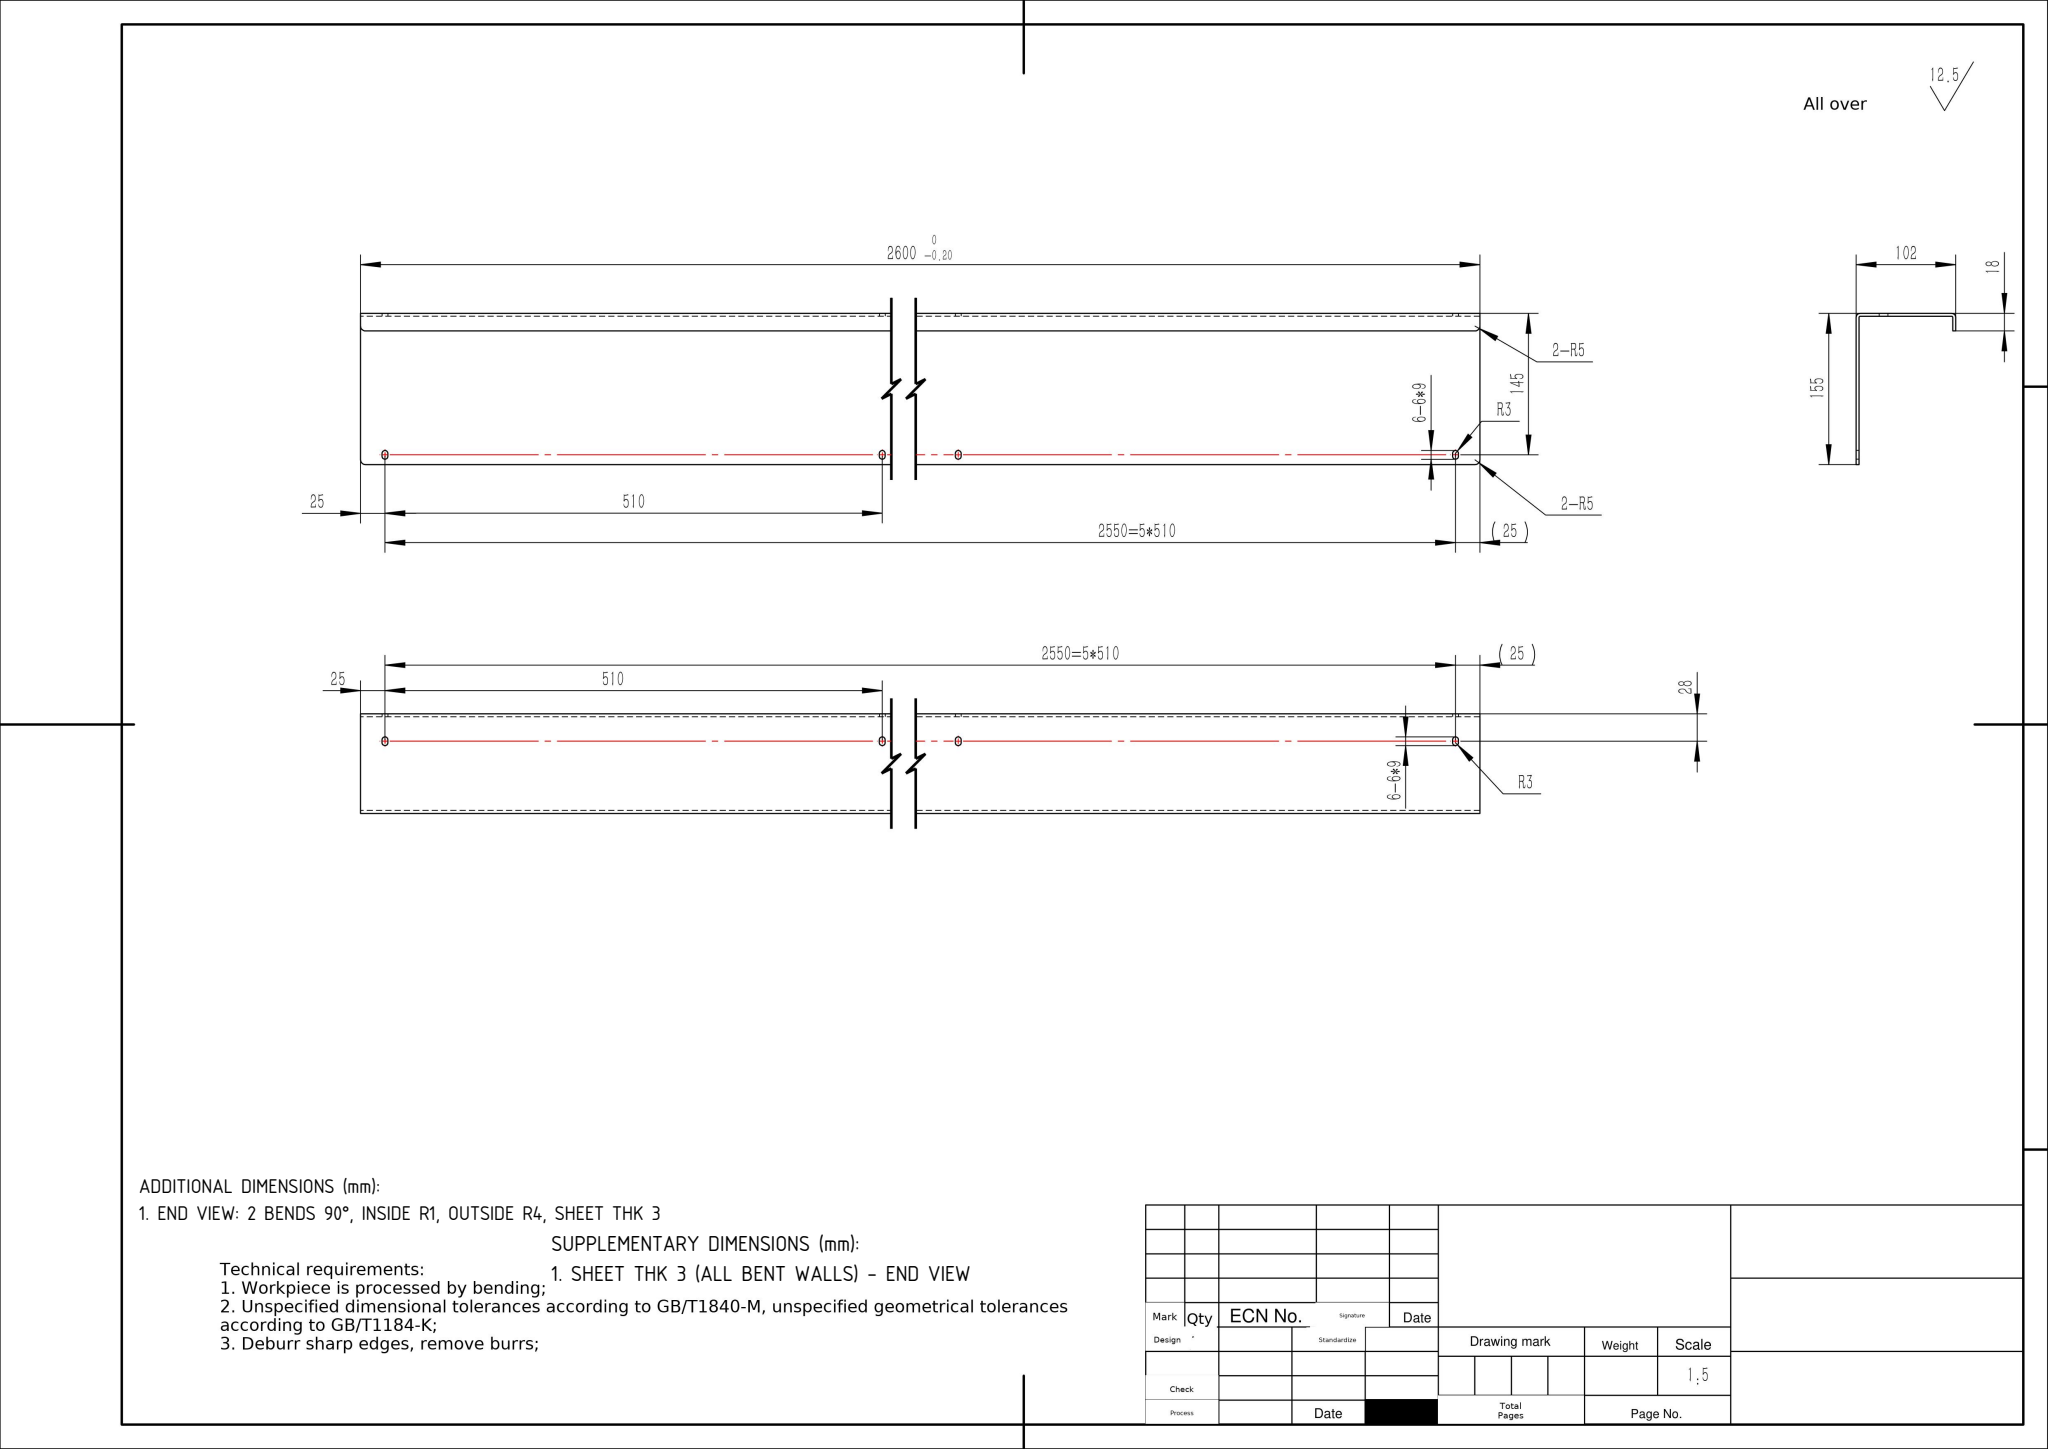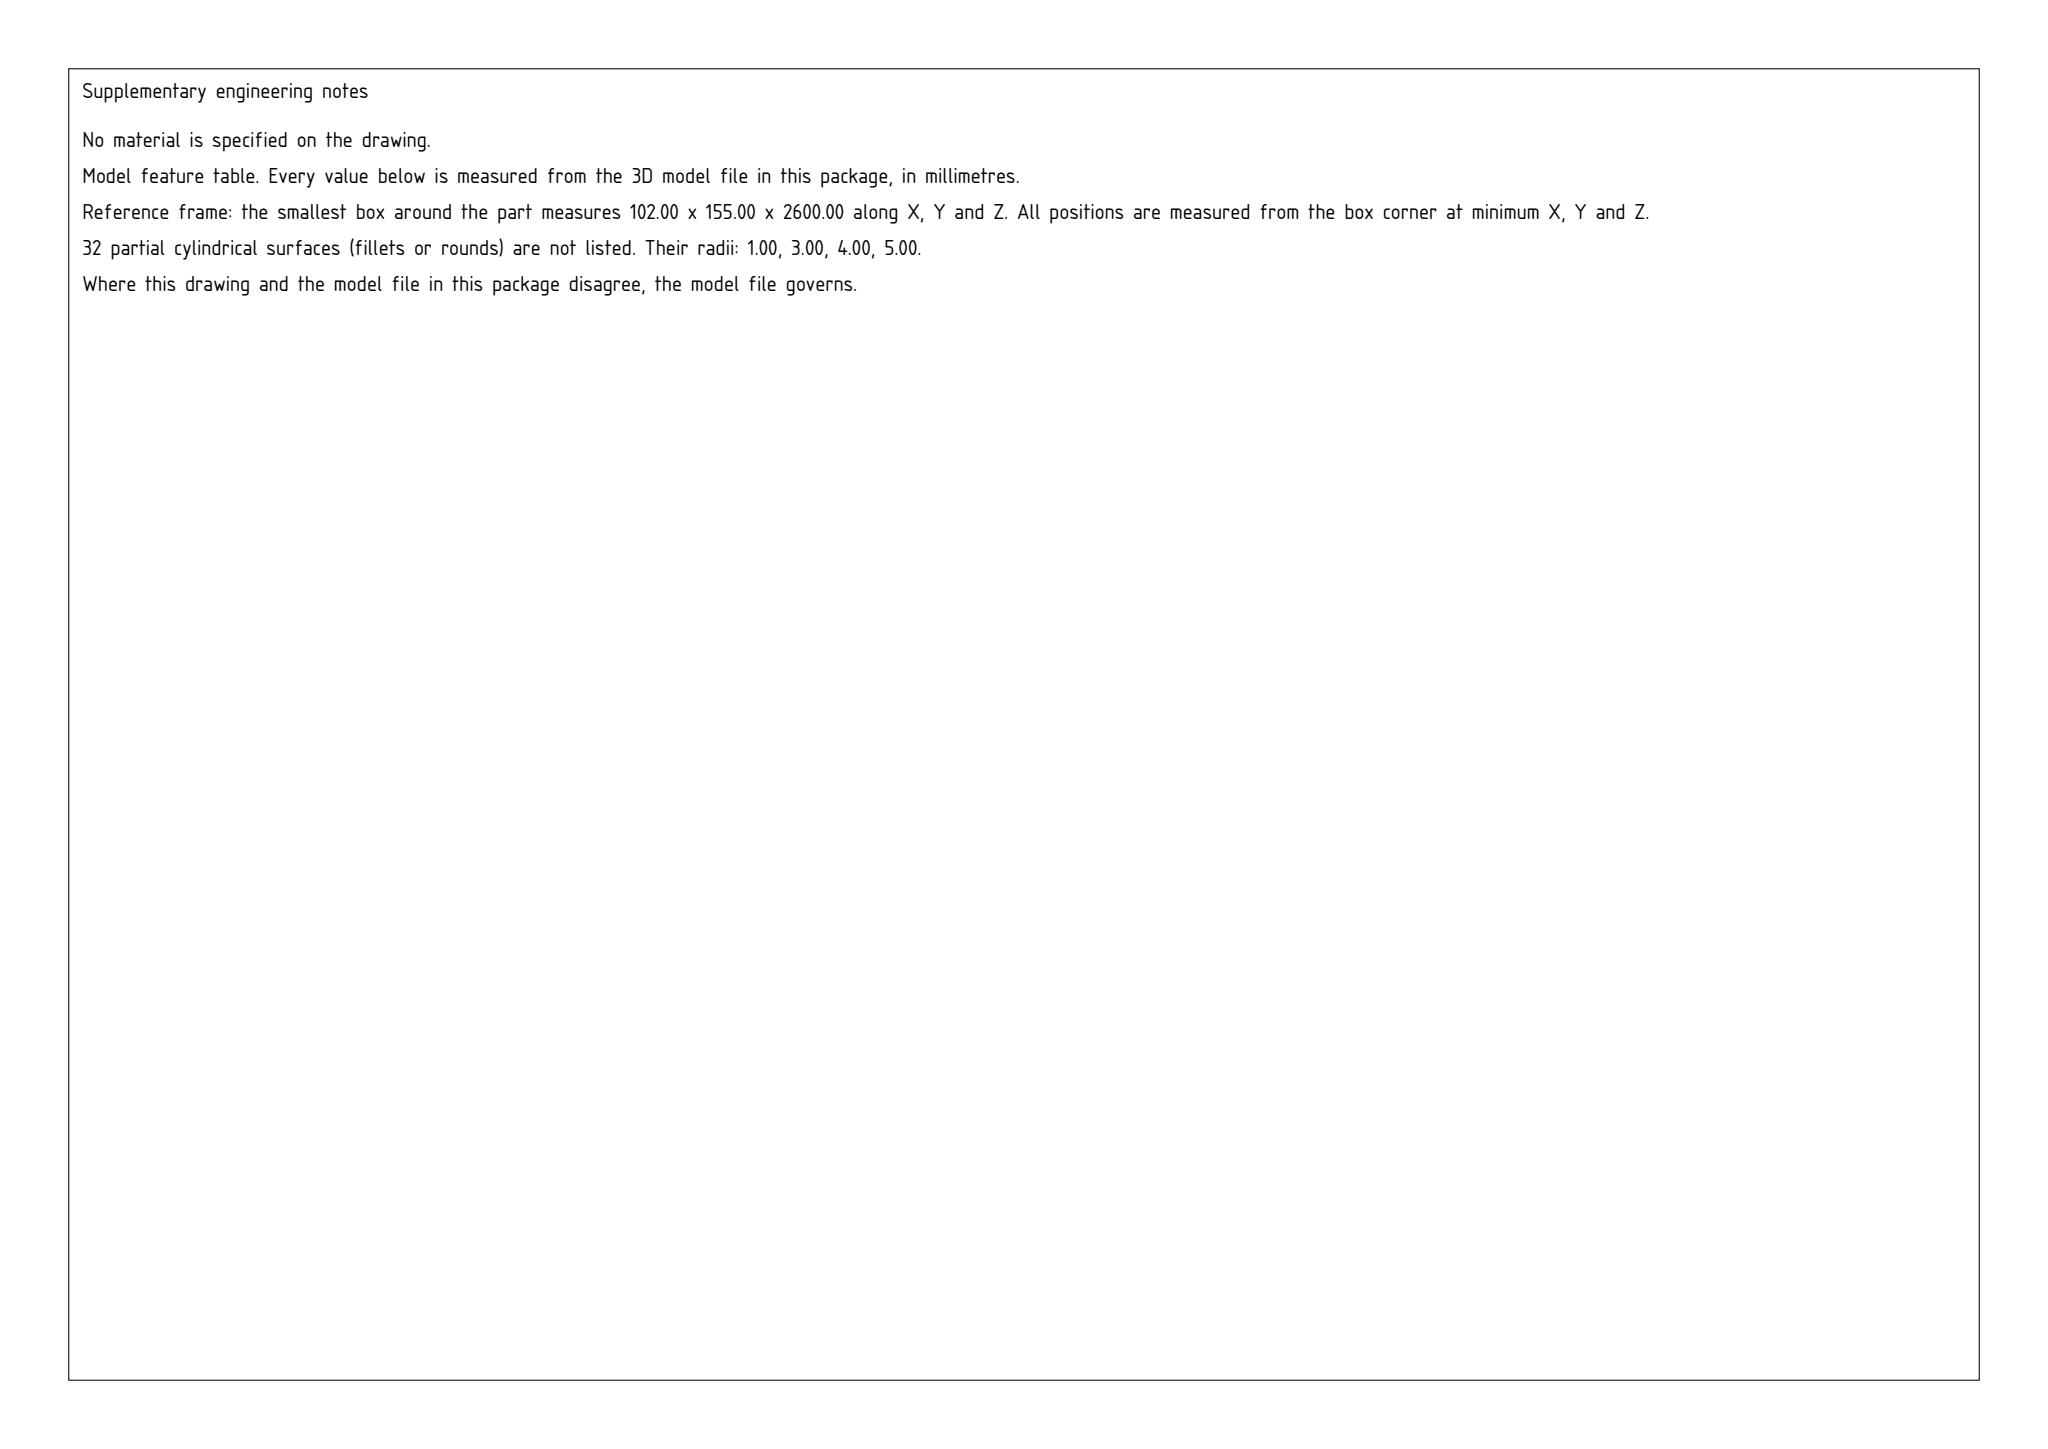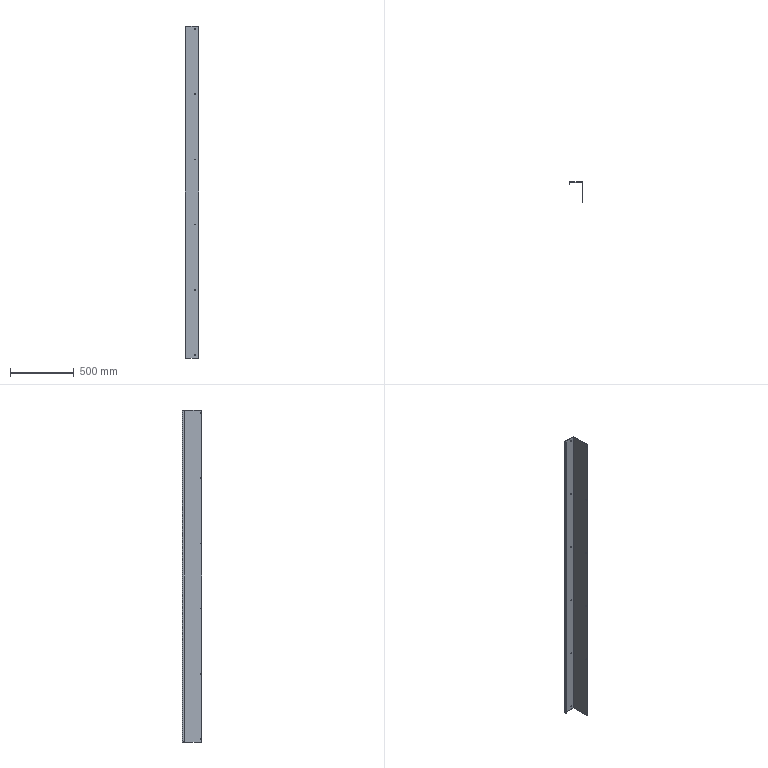Part | SolidWorks | mm | 1 solid | 74 faces | box 102 x 155 x 2600 mm | volume 2079731 mm3 | plane 42 | cylinder 32 | commonest cylinder face diameters 6 x24 10 x4 2 x2 8 x2